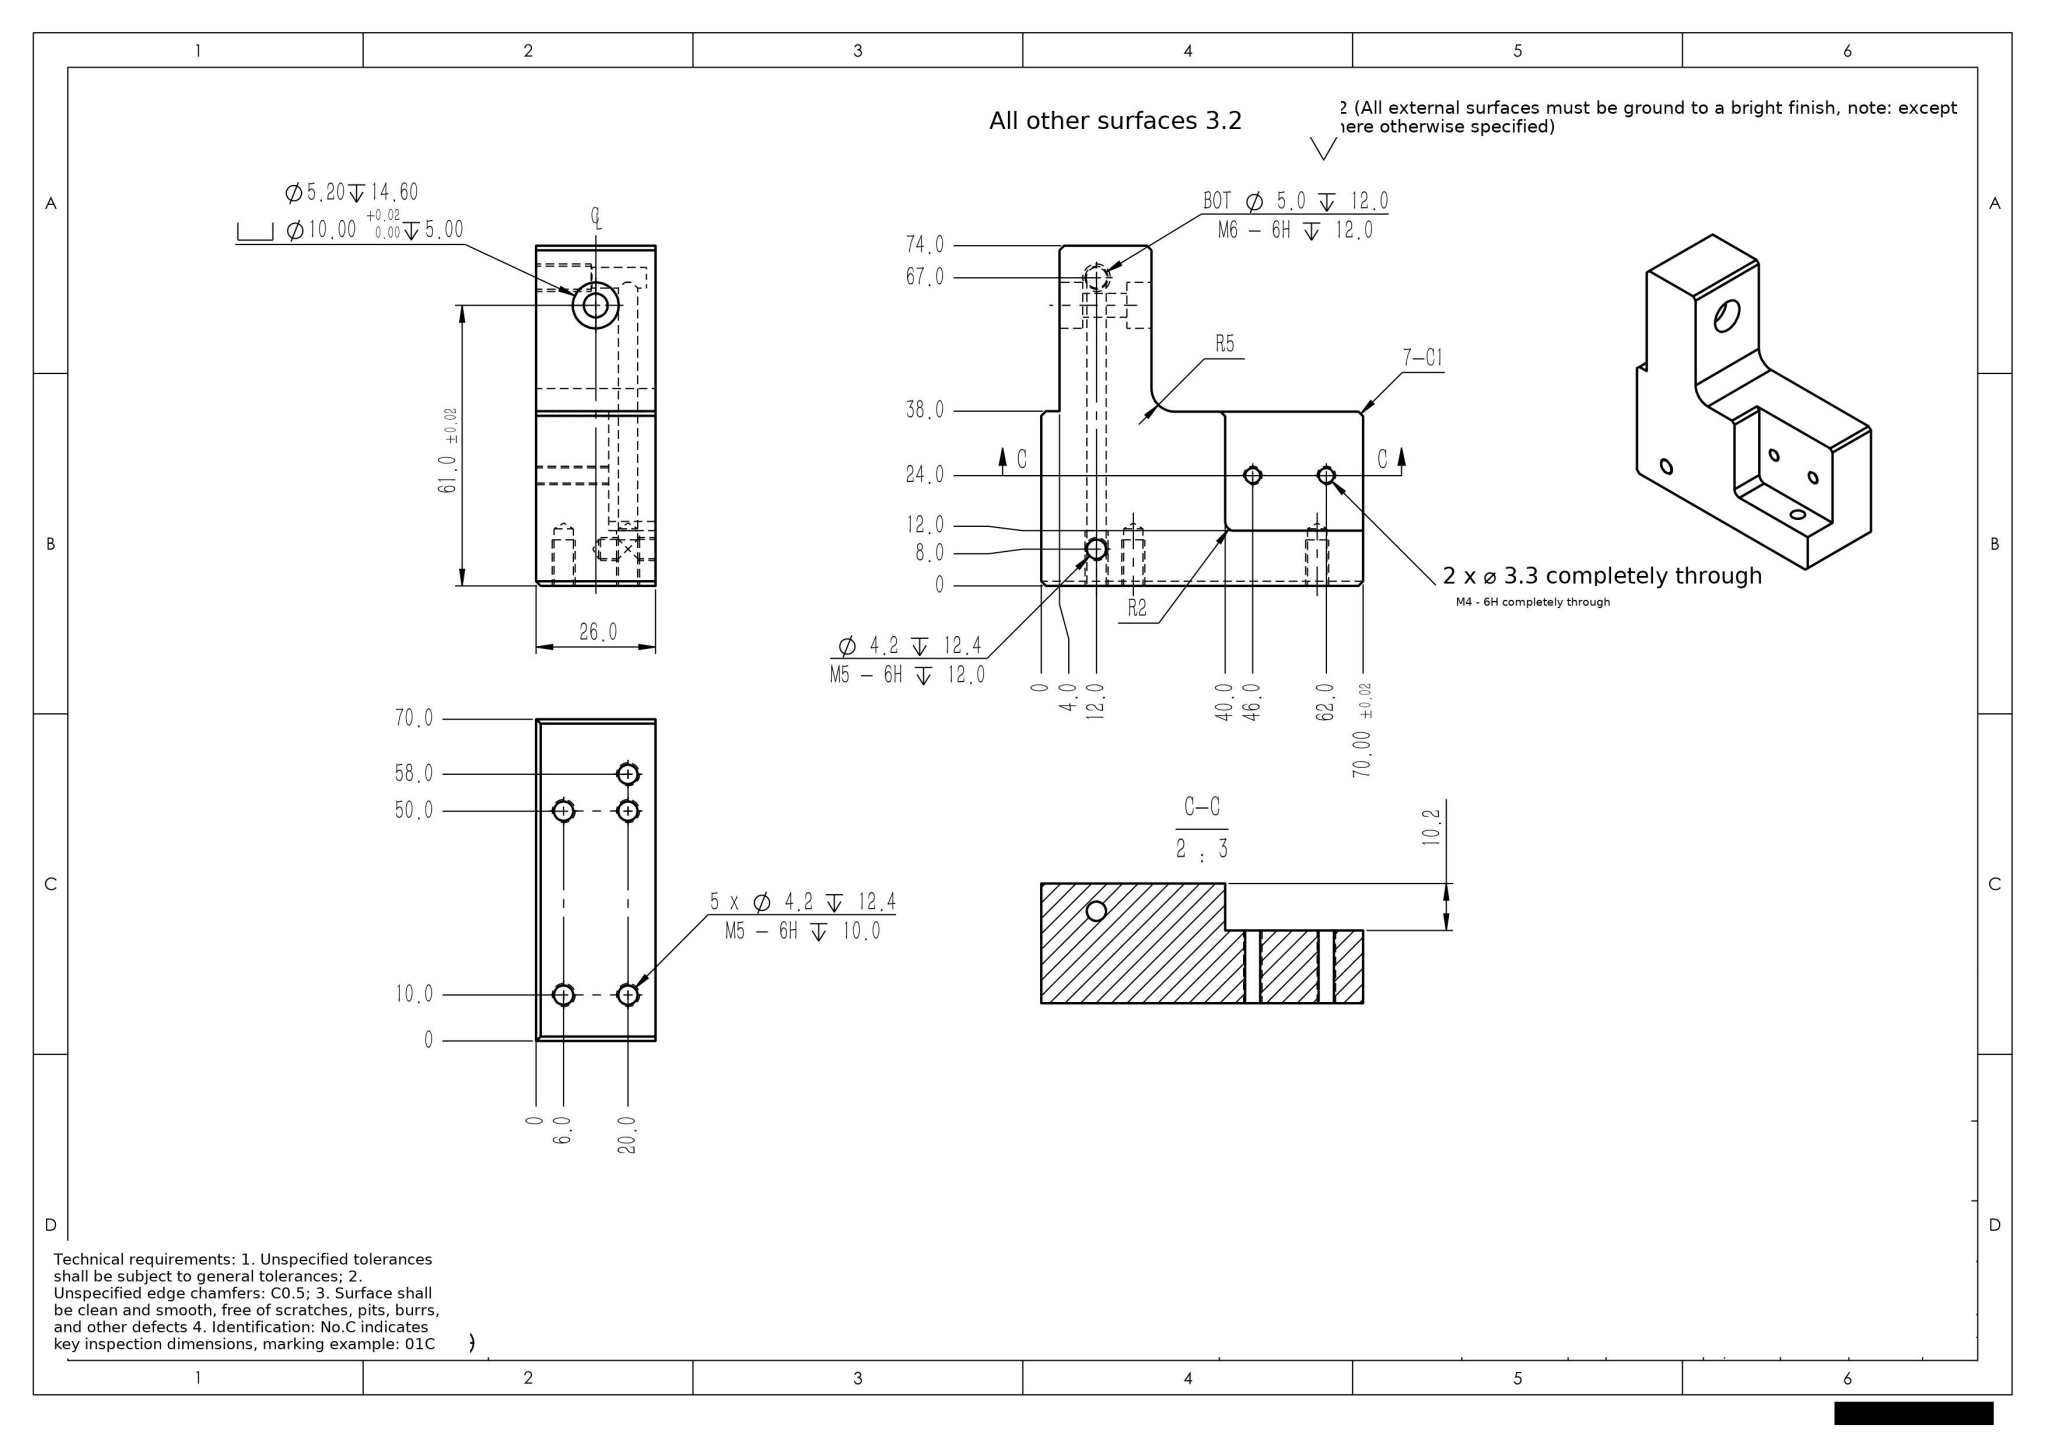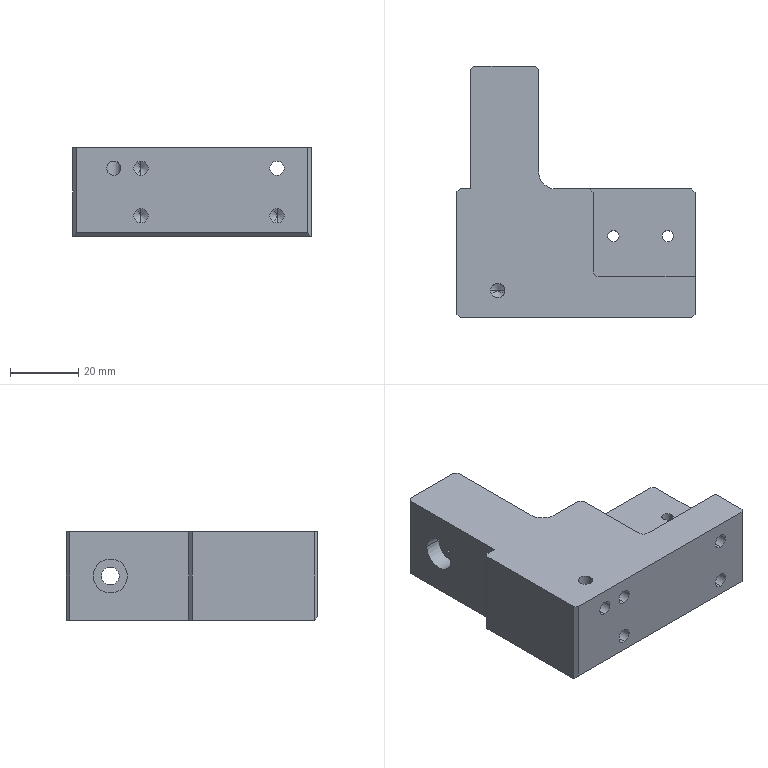Part | SolidWorks | mm | 1 solid | 68 faces | box 70 x 74 x 26 mm | volume 76425 mm3 | cylinder 32 | plane 24 | cone 12 | commonest cylinder face diameters 4.2 x16 10 x5 3.3 x4 4.5 x2 5 x2 5.2 x2 4 x1